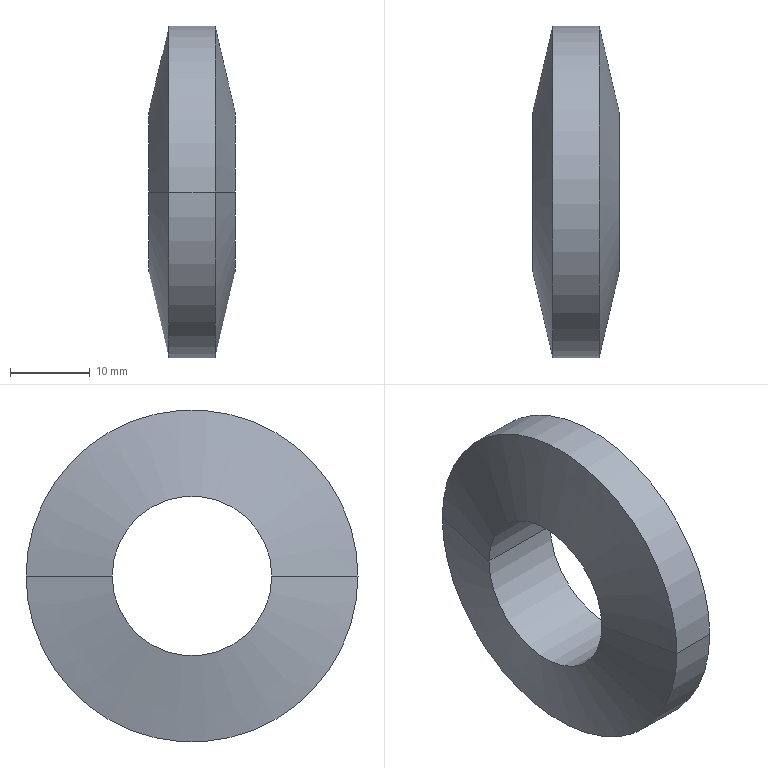Component | SolidWorks | SealingFelt-1 | 1 solid | 8 faces | box 10.82 x 41.57 x 41.57 mm | volume 8363 mm3 | cylinder 4 | cone 4 | commonest cylinder face diameters 20 x2 41.575 x2
build123d program:
from build123d import *


with BuildPart() as part:
    # Sketch2 → Revolve1 (revolve)
    with BuildSketch(Plane(origin=(0, 0, 0), x_dir=(1, 0, 0), z_dir=(0, 1, 0))):
        Polygon((-153.1, 14.233), (-150.592, 25.021), (-161.408, 25.021), (-158.9, 14.233), align=None)
    revolve(axis=Axis((-414, 0, -35.021), (1, 0, 0)))


solid = part.part

# Placed as in the assembly
solid = solid.moved(Location((0, 60.219, 35.021), (0, 0, 0)))
STEP:
#1=COLOUR_RGB('',0.7922,0.8196,0.9333);
#2=FILL_AREA_STYLE_COLOUR('',#1);
#3=FILL_AREA_STYLE('',(#2));
#4=SURFACE_STYLE_FILL_AREA(#3);
#5=SURFACE_SIDE_STYLE('',(#4));
#6=SURFACE_STYLE_USAGE(.BOTH.,#5);
#7=PRESENTATION_STYLE_ASSIGNMENT((#6));
#8=CARTESIAN_POINT('',(-5.929,1.977,-0.));
#9=VERTEX_POINT('',#8);
#10=CARTESIAN_POINT('',(-5.929,2.765,0.));
#11=VERTEX_POINT('',#10);
#12=CARTESIAN_POINT('',(-5.929,2.371,0.));
#13=DIRECTION('',(-1.,0.,0.));
#14=DIRECTION('',(0.,1.,0.));
#15=AXIS2_PLACEMENT_3D('',#12,#13,#14);
#16=CIRCLE('',#15,0.3937);
#17=EDGE_CURVE('',#9,#11,#16,.T.);
#18=ORIENTED_EDGE('',*,*,#17,.F.);
#19=CARTESIAN_POINT('',(-6.355,1.977,0.));
#20=VERTEX_POINT('',#19);
#21=CARTESIAN_POINT('',(-16.299,1.977,-0.));
#22=DIRECTION('',(-1.,0.,0.));
#23=VECTOR('',#22,39.37);
#24=LINE('',#21,#23);
#25=EDGE_CURVE('',#9,#20,#24,.T.);
#26=ORIENTED_EDGE('',*,*,#25,.T.);
#27=CARTESIAN_POINT('',(-6.355,2.765,-0.));
#28=VERTEX_POINT('',#27);
#29=CARTESIAN_POINT('',(-6.355,2.371,0.));
#30=DIRECTION('',(-1.,0.,0.));
#31=DIRECTION('',(0.,1.,0.));
#32=AXIS2_PLACEMENT_3D('',#29,#30,#31);
#33=CIRCLE('',#32,0.3937);
#34=EDGE_CURVE('',#20,#28,#33,.T.);
#35=ORIENTED_EDGE('',*,*,#34,.T.);
#36=CARTESIAN_POINT('',(-16.299,2.765,0.));
#37=DIRECTION('',(-1.,0.,0.));
#38=VECTOR('',#37,39.37);
#39=LINE('',#36,#38);
#40=EDGE_CURVE('',#11,#28,#39,.T.);
#41=ORIENTED_EDGE('',*,*,#40,.F.);
#42=EDGE_LOOP('',(#18,#26,#35,#41));
#43=FACE_OUTER_BOUND('',#42,.T.);
#44=CARTESIAN_POINT('',(-16.299,2.371,0.));
#45=DIRECTION('',(-1.,0.,0.));
#46=DIRECTION('',(0.,1.,0.));
#47=AXIS2_PLACEMENT_3D('',#44,#45,#46);
#48=CYLINDRICAL_SURFACE('',#47,0.3937);
#49=ADVANCED_FACE('',(#43),#48,.F.);
#50=CARTESIAN_POINT('',(-5.929,2.371,0.));
#51=DIRECTION('',(-1.,0.,0.));
#52=DIRECTION('',(0.,1.,0.));
#53=AXIS2_PLACEMENT_3D('',#50,#51,#52);
#54=CIRCLE('',#53,0.3937);
#55=EDGE_CURVE('',#11,#9,#54,.T.);
#56=ORIENTED_EDGE('',*,*,#55,.T.);
#57=CARTESIAN_POINT('',(-6.028,1.552,-0.));
#58=VERTEX_POINT('',#57);
#59=CARTESIAN_POINT('',(-5.929,1.977,-0.));
#60=DIRECTION('',(-0.2264,-0.974,-0.));
#61=VECTOR('',#60,39.37);
#62=LINE('',#59,#61);
#63=EDGE_CURVE('',#9,#58,#62,.T.);
#64=ORIENTED_EDGE('',*,*,#63,.T.);
#65=CARTESIAN_POINT('',(-6.028,3.189,0.));
#66=VERTEX_POINT('',#65);
#67=CARTESIAN_POINT('',(-6.028,2.371,0.));
#68=DIRECTION('',(-1.,0.,0.));
#69=DIRECTION('',(0.,1.,0.));
#70=AXIS2_PLACEMENT_3D('',#67,#68,#69);
#71=CIRCLE('',#70,0.8184);
#72=EDGE_CURVE('',#66,#58,#71,.T.);
#73=ORIENTED_EDGE('',*,*,#72,.F.);
#74=CARTESIAN_POINT('',(-5.929,2.765,0.));
#75=DIRECTION('',(-0.2264,0.974,0.));
#76=VECTOR('',#75,39.37);
#77=LINE('',#74,#76);
#78=EDGE_CURVE('',#11,#66,#77,.T.);
#79=ORIENTED_EDGE('',*,*,#78,.F.);
#80=EDGE_LOOP('',(#56,#64,#73,#79));
#81=FACE_OUTER_BOUND('',#80,.T.);
#82=CARTESIAN_POINT('',(-5.929,2.371,0.));
#83=DIRECTION('',(-1.,0.,0.));
#84=DIRECTION('',(0.,1.,0.));
#85=AXIS2_PLACEMENT_3D('',#82,#83,#84);
#86=CONICAL_SURFACE('',#85,0.3937,1.342);
#87=ADVANCED_FACE('',(#81),#86,.T.);
#88=ORIENTED_EDGE('',*,*,#72,.T.);
#89=CARTESIAN_POINT('',(-6.256,1.552,0.));
#90=VERTEX_POINT('',#89);
#91=CARTESIAN_POINT('',(-16.299,1.552,-0.));
#92=DIRECTION('',(-1.,0.,0.));
#93=VECTOR('',#92,39.37);
#94=LINE('',#91,#93);
#95=EDGE_CURVE('',#58,#90,#94,.T.);
#96=ORIENTED_EDGE('',*,*,#95,.T.);
#97=CARTESIAN_POINT('',(-6.256,3.189,-0.));
#98=VERTEX_POINT('',#97);
#99=CARTESIAN_POINT('',(-6.256,2.371,0.));
#100=DIRECTION('',(-1.,0.,0.));
#101=DIRECTION('',(0.,1.,0.));
#102=AXIS2_PLACEMENT_3D('',#99,#100,#101);
#103=CIRCLE('',#102,0.8184);
#104=EDGE_CURVE('',#98,#90,#103,.T.);
#105=ORIENTED_EDGE('',*,*,#104,.F.);
#106=CARTESIAN_POINT('',(-16.299,3.189,0.));
#107=DIRECTION('',(-1.,0.,0.));
#108=VECTOR('',#107,39.37);
#109=LINE('',#106,#108);
#110=EDGE_CURVE('',#66,#98,#109,.T.);
#111=ORIENTED_EDGE('',*,*,#110,.F.);
#112=EDGE_LOOP('',(#88,#96,#105,#111));
#113=FACE_OUTER_BOUND('',#112,.T.);
#114=CARTESIAN_POINT('',(-16.299,2.371,0.));
#115=DIRECTION('',(-1.,0.,0.));
#116=DIRECTION('',(0.,1.,0.));
#117=AXIS2_PLACEMENT_3D('',#114,#115,#116);
#118=CYLINDRICAL_SURFACE('',#117,0.8184);
#119=ADVANCED_FACE('',(#113),#118,.T.);
#120=CARTESIAN_POINT('',(-6.355,2.371,0.));
#121=DIRECTION('',(-1.,0.,0.));
#122=DIRECTION('',(0.,1.,0.));
#123=AXIS2_PLACEMENT_3D('',#120,#121,#122);
#124=CIRCLE('',#123,0.3937);
#125=EDGE_CURVE('',#28,#20,#124,.T.);
#126=ORIENTED_EDGE('',*,*,#125,.F.);
#127=CARTESIAN_POINT('',(-6.355,2.765,-0.));
#128=DIRECTION('',(0.2264,0.974,-0.));
#129=VECTOR('',#128,39.37);
#130=LINE('',#127,#129);
#131=EDGE_CURVE('',#28,#98,#130,.T.);
#132=ORIENTED_EDGE('',*,*,#131,.T.);
#133=ORIENTED_EDGE('',*,*,#104,.T.);
#134=CARTESIAN_POINT('',(-6.355,1.977,0.));
#135=DIRECTION('',(0.2264,-0.974,0.));
#136=VECTOR('',#135,39.37);
#137=LINE('',#134,#136);
#138=EDGE_CURVE('',#20,#90,#137,.T.);
#139=ORIENTED_EDGE('',*,*,#138,.F.);
#140=EDGE_LOOP('',(#126,#132,#133,#139));
#141=FACE_OUTER_BOUND('',#140,.T.);
#142=CARTESIAN_POINT('',(-6.355,2.371,0.));
#143=DIRECTION('',(1.,0.,0.));
#144=DIRECTION('',(0.,-1.,0.));
#145=AXIS2_PLACEMENT_3D('',#142,#143,#144);
#146=CONICAL_SURFACE('',#145,0.3937,1.342);
#147=ADVANCED_FACE('',(#141),#146,.T.);
#148=ORIENTED_EDGE('',*,*,#131,.F.);
#149=ORIENTED_EDGE('',*,*,#34,.F.);
#150=ORIENTED_EDGE('',*,*,#138,.T.);
#151=CARTESIAN_POINT('',(-6.256,2.371,0.));
#152=DIRECTION('',(-1.,0.,0.));
#153=DIRECTION('',(0.,1.,0.));
#154=AXIS2_PLACEMENT_3D('',#151,#152,#153);
#155=CIRCLE('',#154,0.8184);
#156=EDGE_CURVE('',#90,#98,#155,.T.);
#157=ORIENTED_EDGE('',*,*,#156,.T.);
#158=EDGE_LOOP('',(#148,#149,#150,#157));
#159=FACE_OUTER_BOUND('',#158,.T.);
#160=CARTESIAN_POINT('',(-6.355,2.371,0.));
#161=DIRECTION('',(1.,0.,0.));
#162=DIRECTION('',(0.,-1.,0.));
#163=AXIS2_PLACEMENT_3D('',#160,#161,#162);
#164=CONICAL_SURFACE('',#163,0.3937,1.342);
#165=ADVANCED_FACE('',(#159),#164,.T.);
#166=ORIENTED_EDGE('',*,*,#95,.F.);
#167=CARTESIAN_POINT('',(-6.028,2.371,0.));
#168=DIRECTION('',(-1.,0.,0.));
#169=DIRECTION('',(0.,1.,0.));
#170=AXIS2_PLACEMENT_3D('',#167,#168,#169);
#171=CIRCLE('',#170,0.8184);
#172=EDGE_CURVE('',#58,#66,#171,.T.);
#173=ORIENTED_EDGE('',*,*,#172,.T.);
#174=ORIENTED_EDGE('',*,*,#110,.T.);
#175=ORIENTED_EDGE('',*,*,#156,.F.);
#176=EDGE_LOOP('',(#166,#173,#174,#175));
#177=FACE_OUTER_BOUND('',#176,.T.);
#178=CARTESIAN_POINT('',(-16.299,2.371,0.));
#179=DIRECTION('',(-1.,0.,0.));
#180=DIRECTION('',(0.,1.,0.));
#181=AXIS2_PLACEMENT_3D('',#178,#179,#180);
#182=CYLINDRICAL_SURFACE('',#181,0.8184);
#183=ADVANCED_FACE('',(#177),#182,.T.);
#184=ORIENTED_EDGE('',*,*,#63,.F.);
#185=ORIENTED_EDGE('',*,*,#17,.T.);
#186=ORIENTED_EDGE('',*,*,#78,.T.);
#187=ORIENTED_EDGE('',*,*,#172,.F.);
#188=EDGE_LOOP('',(#184,#185,#186,#187));
#189=FACE_OUTER_BOUND('',#188,.T.);
#190=CARTESIAN_POINT('',(-5.929,2.371,0.));
#191=DIRECTION('',(-1.,0.,0.));
#192=DIRECTION('',(0.,1.,0.));
#193=AXIS2_PLACEMENT_3D('',#190,#191,#192);
#194=CONICAL_SURFACE('',#193,0.3937,1.342);
#195=ADVANCED_FACE('',(#189),#194,.T.);
#196=ORIENTED_EDGE('',*,*,#25,.F.);
#197=ORIENTED_EDGE('',*,*,#55,.F.);
#198=ORIENTED_EDGE('',*,*,#40,.T.);
#199=ORIENTED_EDGE('',*,*,#125,.T.);
#200=EDGE_LOOP('',(#196,#197,#198,#199));
#201=FACE_OUTER_BOUND('',#200,.T.);
#202=CARTESIAN_POINT('',(-16.299,2.371,0.));
#203=DIRECTION('',(-1.,0.,0.));
#204=DIRECTION('',(0.,1.,0.));
#205=AXIS2_PLACEMENT_3D('',#202,#203,#204);
#206=CYLINDRICAL_SURFACE('',#205,0.3937);
#207=ADVANCED_FACE('',(#201),#206,.F.);
#208=CLOSED_SHELL('',(#49,#87,#119,#147,#165,#183,#195,#207));
#209=MANIFOLD_SOLID_BREP('',#208);
#210=STYLED_ITEM('',(#7),#209);
#211=PRESENTATION_LAYER_ASSIGNMENT('','',(#210));
#212=(LENGTH_UNIT()NAMED_UNIT(*)SI_UNIT($,.METRE.));
#213=LENGTH_MEASURE_WITH_UNIT(LENGTH_MEASURE(0.0254),#212);
#214=DIMENSIONAL_EXPONENTS(1.,0.,0.,0.,0.,0.,0.);
#215=(CONVERSION_BASED_UNIT('',#213)LENGTH_UNIT()NAMED_UNIT(#214));
#216=UNCERTAINTY_MEASURE_WITH_UNIT(LENGTH_MEASURE(0.00001),#215,'','');
#217=(NAMED_UNIT(*)PLANE_ANGLE_UNIT()SI_UNIT($,.RADIAN.));
#218=(NAMED_UNIT(*)SI_UNIT($,.STERADIAN.)SOLID_ANGLE_UNIT());
#219=(GEOMETRIC_REPRESENTATION_CONTEXT(3)GLOBAL_UNCERTAINTY_ASSIGNED_CONTEXT((#216))GLOBAL_UNIT_ASSIGNED_CONTEXT((#215,#217,#218))REPRESENTATION_CONTEXT('',''));
#220=MECHANICAL_DESIGN_GEOMETRIC_PRESENTATION_REPRESENTATION('',(#210),#219);
#221=CARTESIAN_POINT('',(0.,0.,0.));
#222=DIRECTION('',(0.,0.,1.));
#223=DIRECTION('',(1.,0.,0.));
#224=AXIS2_PLACEMENT_3D('',#221,#222,#223);
#225=(LENGTH_UNIT()NAMED_UNIT(*)SI_UNIT($,.METRE.));
#226=LENGTH_MEASURE_WITH_UNIT(LENGTH_MEASURE(0.0254),#225);
#227=DIMENSIONAL_EXPONENTS(1.,0.,0.,0.,0.,0.,0.);
#228=(CONVERSION_BASED_UNIT('',#226)LENGTH_UNIT()NAMED_UNIT(#227));
#229=UNCERTAINTY_MEASURE_WITH_UNIT(LENGTH_MEASURE(0.00001),#228,'','');
#230=(NAMED_UNIT(*)PLANE_ANGLE_UNIT()SI_UNIT($,.RADIAN.));
#231=(NAMED_UNIT(*)SI_UNIT($,.STERADIAN.)SOLID_ANGLE_UNIT());
#232=(GEOMETRIC_REPRESENTATION_CONTEXT(3)GLOBAL_UNCERTAINTY_ASSIGNED_CONTEXT((#229))GLOBAL_UNIT_ASSIGNED_CONTEXT((#228,#230,#231))REPRESENTATION_CONTEXT('',''));
#233=ADVANCED_BREP_SHAPE_REPRESENTATION('',(#209,#224),#232);